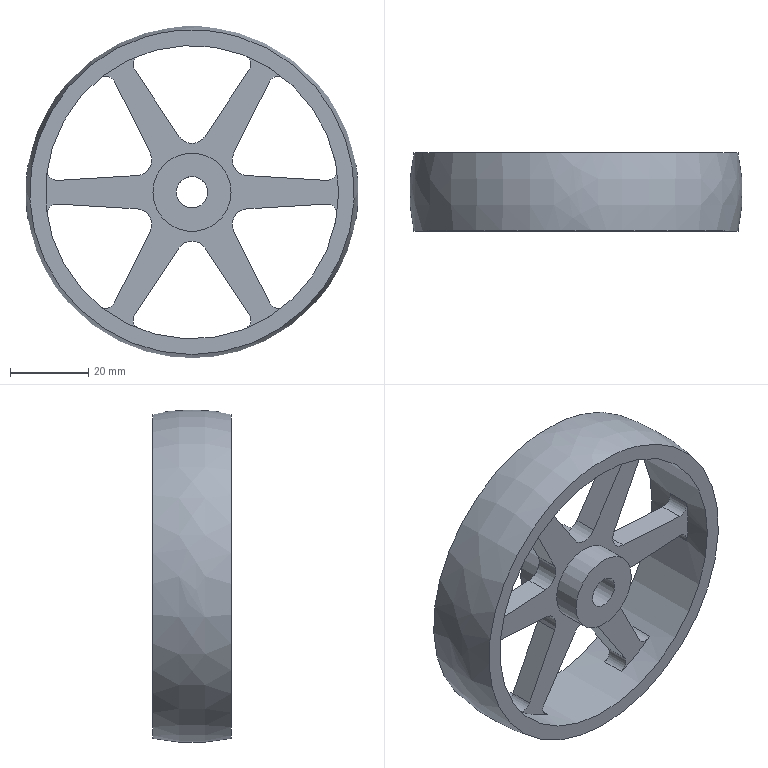Component | NX | SMALL_FLYWHEEL | 1 solid | 41 faces | volume 36397 mm3 | cylinder 22 | plane 18 | spline 1 | commonest cylinder face diameters 5 x12 8 x7 20 x2 75 x1